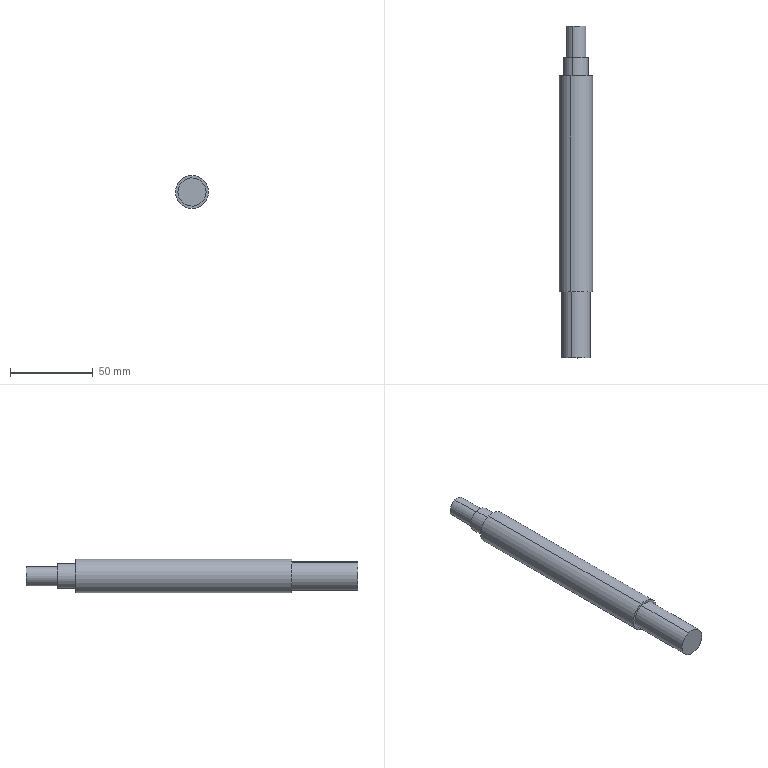Component | SolidWorks | CenterAxis-1 | 1 solid | 13 faces | box 20 x 200 x 20 mm | volume 54013 mm3 | cylinder 8 | plane 5 | commonest cylinder face diameters 12 x2 15 x2 20 x2 17 x2
build123d program:
from build123d import *

# Parameters (mm, degrees)
SKETCH2_R      = 7.5
EXTRUDE1_DEPTH = 11


with BuildPart() as part:
    # Sketch1 → Revolve1 (revolve)
    with BuildSketch(Plane.XY, mode=Mode.PRIVATE) as revolve1_sk:
        Polygon((0, 86.08), (8.5, 86.08), (8.5, 46.08), (10, 46.08), (10, -83.92), (6, -83.92), (6, -113.92), (0, -113.92), align=None)
    revolve(revolve1_sk.sketch.rotate(Axis((0, 0, 0), (0, 1, 0)), 90), axis=Axis((0, 0, 0), (0, 1, 0)))

    # Sketch2 → Extrude1 (add)
    with BuildSketch(Plane.XZ.offset(83.92)):
        with Locations(Location((0, 0, 0), (0, 0, 270))):
            Circle(SKETCH2_R)
    extrude(amount=EXTRUDE1_DEPTH)


solid = part.part

# Placed as in the assembly
solid = solid.moved(Location((-164.784, 362.063, 4), (180, 0, 0)))
STEP:
#1=COLOUR_RGB('',0.7922,0.8196,0.9333);
#2=FILL_AREA_STYLE_COLOUR('',#1);
#3=FILL_AREA_STYLE('',(#2));
#4=SURFACE_STYLE_FILL_AREA(#3);
#5=SURFACE_SIDE_STYLE('',(#4));
#6=SURFACE_STYLE_USAGE(.BOTH.,#5);
#7=PRESENTATION_STYLE_ASSIGNMENT((#6));
#8=CARTESIAN_POINT('',(-6.563,17.991,0.3814));
#9=VERTEX_POINT('',#8);
#10=CARTESIAN_POINT('',(-6.412,17.991,-0.06641));
#11=VERTEX_POINT('',#10);
#12=CARTESIAN_POINT('',(-6.488,17.991,0.1575));
#13=DIRECTION('',(0.,-1.,0.));
#14=DIRECTION('',(0.3188,0.,-0.9478));
#15=AXIS2_PLACEMENT_3D('',#12,#13,#14);
#16=CIRCLE('',#15,0.2362);
#17=EDGE_CURVE('',#9,#11,#16,.T.);
#18=ORIENTED_EDGE('',*,*,#17,.F.);
#19=CARTESIAN_POINT('',(-6.563,18.74,0.3814));
#20=VERTEX_POINT('',#19);
#21=CARTESIAN_POINT('',(-6.563,14.254,0.3814));
#22=DIRECTION('',(-0.,1.,-0.));
#23=VECTOR('',#22,39.37);
#24=LINE('',#21,#23);
#25=EDGE_CURVE('',#9,#20,#24,.T.);
#26=ORIENTED_EDGE('',*,*,#25,.T.);
#27=CARTESIAN_POINT('',(-6.412,18.74,-0.06641));
#28=VERTEX_POINT('',#27);
#29=CARTESIAN_POINT('',(-6.488,18.74,0.1575));
#30=DIRECTION('',(-0.,1.,-0.));
#31=DIRECTION('',(0.3188,0.,-0.9478));
#32=AXIS2_PLACEMENT_3D('',#29,#30,#31);
#33=CIRCLE('',#32,0.2362);
#34=EDGE_CURVE('',#28,#20,#33,.T.);
#35=ORIENTED_EDGE('',*,*,#34,.F.);
#36=CARTESIAN_POINT('',(-6.412,14.254,-0.06641));
#37=DIRECTION('',(-0.,1.,-0.));
#38=VECTOR('',#37,39.37);
#39=LINE('',#36,#38);
#40=EDGE_CURVE('',#11,#28,#39,.T.);
#41=ORIENTED_EDGE('',*,*,#40,.F.);
#42=EDGE_LOOP('',(#18,#26,#35,#41));
#43=FACE_OUTER_BOUND('',#42,.T.);
#44=CARTESIAN_POINT('',(-6.488,14.254,0.1575));
#45=DIRECTION('',(-0.,1.,-0.));
#46=DIRECTION('',(0.3188,0.,-0.9478));
#47=AXIS2_PLACEMENT_3D('',#44,#45,#46);
#48=CYLINDRICAL_SURFACE('',#47,0.2362);
#49=ADVANCED_FACE('',(#43),#48,.T.);
#50=CARTESIAN_POINT('',(-6.393,17.991,-0.1224));
#51=VERTEX_POINT('',#50);
#52=CARTESIAN_POINT('',(-6.582,17.991,0.4373));
#53=VERTEX_POINT('',#52);
#54=CARTESIAN_POINT('',(-6.488,17.991,0.1575));
#55=DIRECTION('',(-0.,1.,-0.));
#56=DIRECTION('',(0.3188,0.,-0.9478));
#57=AXIS2_PLACEMENT_3D('',#54,#55,#56);
#58=CIRCLE('',#57,0.2953);
#59=EDGE_CURVE('',#51,#53,#58,.T.);
#60=ORIENTED_EDGE('',*,*,#59,.F.);
#61=CARTESIAN_POINT('',(-6.393,17.558,-0.1224));
#62=VERTEX_POINT('',#61);
#63=CARTESIAN_POINT('',(-6.393,17.991,-0.1224));
#64=DIRECTION('',(0.,-1.,0.));
#65=VECTOR('',#64,39.37);
#66=LINE('',#63,#65);
#67=EDGE_CURVE('',#51,#62,#66,.T.);
#68=ORIENTED_EDGE('',*,*,#67,.T.);
#69=CARTESIAN_POINT('',(-6.582,17.558,0.4373));
#70=VERTEX_POINT('',#69);
#71=CARTESIAN_POINT('',(-6.488,17.558,0.1575));
#72=DIRECTION('',(-0.,1.,-0.));
#73=DIRECTION('',(0.3188,0.,-0.9478));
#74=AXIS2_PLACEMENT_3D('',#71,#72,#73);
#75=CIRCLE('',#74,0.2953);
#76=EDGE_CURVE('',#62,#70,#75,.T.);
#77=ORIENTED_EDGE('',*,*,#76,.T.);
#78=CARTESIAN_POINT('',(-6.582,17.991,0.4373));
#79=DIRECTION('',(0.,-1.,0.));
#80=VECTOR('',#79,39.37);
#81=LINE('',#78,#80);
#82=EDGE_CURVE('',#53,#70,#81,.T.);
#83=ORIENTED_EDGE('',*,*,#82,.F.);
#84=EDGE_LOOP('',(#60,#68,#77,#83));
#85=FACE_OUTER_BOUND('',#84,.T.);
#86=CARTESIAN_POINT('',(-6.488,17.991,0.1575));
#87=DIRECTION('',(0.,-1.,0.));
#88=DIRECTION('',(-0.3188,0.,0.9478));
#89=AXIS2_PLACEMENT_3D('',#86,#87,#88);
#90=CYLINDRICAL_SURFACE('',#89,0.2953);
#91=ADVANCED_FACE('',(#85),#90,.T.);
#92=CARTESIAN_POINT('',(-6.362,12.44,-0.2157));
#93=VERTEX_POINT('',#92);
#94=CARTESIAN_POINT('',(-6.613,12.44,0.5306));
#95=VERTEX_POINT('',#94);
#96=CARTESIAN_POINT('',(-6.488,12.44,0.1575));
#97=DIRECTION('',(-0.,1.,-0.));
#98=DIRECTION('',(0.3188,0.,-0.9478));
#99=AXIS2_PLACEMENT_3D('',#96,#97,#98);
#100=CIRCLE('',#99,0.3937);
#101=EDGE_CURVE('',#93,#95,#100,.T.);
#102=ORIENTED_EDGE('',*,*,#101,.T.);
#103=CARTESIAN_POINT('',(-6.613,17.558,0.5306));
#104=VERTEX_POINT('',#103);
#105=CARTESIAN_POINT('',(-6.613,14.254,0.5306));
#106=DIRECTION('',(-0.,1.,-0.));
#107=VECTOR('',#106,39.37);
#108=LINE('',#105,#107);
#109=EDGE_CURVE('',#95,#104,#108,.T.);
#110=ORIENTED_EDGE('',*,*,#109,.T.);
#111=CARTESIAN_POINT('',(-6.362,17.558,-0.2157));
#112=VERTEX_POINT('',#111);
#113=CARTESIAN_POINT('',(-6.488,17.558,0.1575));
#114=DIRECTION('',(-0.,1.,-0.));
#115=DIRECTION('',(0.3188,0.,-0.9478));
#116=AXIS2_PLACEMENT_3D('',#113,#114,#115);
#117=CIRCLE('',#116,0.3937);
#118=EDGE_CURVE('',#112,#104,#117,.T.);
#119=ORIENTED_EDGE('',*,*,#118,.F.);
#120=CARTESIAN_POINT('',(-6.362,14.254,-0.2157));
#121=DIRECTION('',(-0.,1.,-0.));
#122=VECTOR('',#121,39.37);
#123=LINE('',#120,#122);
#124=EDGE_CURVE('',#93,#112,#123,.T.);
#125=ORIENTED_EDGE('',*,*,#124,.F.);
#126=EDGE_LOOP('',(#102,#110,#119,#125));
#127=FACE_OUTER_BOUND('',#126,.T.);
#128=CARTESIAN_POINT('',(-6.488,14.254,0.1575));
#129=DIRECTION('',(-0.,1.,-0.));
#130=DIRECTION('',(0.3188,0.,-0.9478));
#131=AXIS2_PLACEMENT_3D('',#128,#129,#130);
#132=CYLINDRICAL_SURFACE('',#131,0.3937);
#133=ADVANCED_FACE('',(#127),#132,.T.);
#134=CARTESIAN_POINT('',(-6.381,10.865,-0.1597));
#135=VERTEX_POINT('',#134);
#136=CARTESIAN_POINT('',(-6.594,10.865,0.4747));
#137=VERTEX_POINT('',#136);
#138=CARTESIAN_POINT('',(-6.488,10.865,0.1575));
#139=DIRECTION('',(-0.,1.,-0.));
#140=DIRECTION('',(0.3188,0.,-0.9478));
#141=AXIS2_PLACEMENT_3D('',#138,#139,#140);
#142=CIRCLE('',#141,0.3346);
#143=EDGE_CURVE('',#135,#137,#142,.T.);
#144=ORIENTED_EDGE('',*,*,#143,.T.);
#145=CARTESIAN_POINT('',(-6.594,12.44,0.4747));
#146=VERTEX_POINT('',#145);
#147=CARTESIAN_POINT('',(-6.594,14.254,0.4747));
#148=DIRECTION('',(-0.,1.,-0.));
#149=VECTOR('',#148,39.37);
#150=LINE('',#147,#149);
#151=EDGE_CURVE('',#137,#146,#150,.T.);
#152=ORIENTED_EDGE('',*,*,#151,.T.);
#153=CARTESIAN_POINT('',(-6.381,12.44,-0.1597));
#154=VERTEX_POINT('',#153);
#155=CARTESIAN_POINT('',(-6.488,12.44,0.1575));
#156=DIRECTION('',(-0.,1.,-0.));
#157=DIRECTION('',(0.3188,0.,-0.9478));
#158=AXIS2_PLACEMENT_3D('',#155,#156,#157);
#159=CIRCLE('',#158,0.3346);
#160=EDGE_CURVE('',#154,#146,#159,.T.);
#161=ORIENTED_EDGE('',*,*,#160,.F.);
#162=CARTESIAN_POINT('',(-6.381,14.254,-0.1597));
#163=DIRECTION('',(-0.,1.,-0.));
#164=VECTOR('',#163,39.37);
#165=LINE('',#162,#164);
#166=EDGE_CURVE('',#135,#154,#165,.T.);
#167=ORIENTED_EDGE('',*,*,#166,.F.);
#168=EDGE_LOOP('',(#144,#152,#161,#167));
#169=FACE_OUTER_BOUND('',#168,.T.);
#170=CARTESIAN_POINT('',(-6.488,14.254,0.1575));
#171=DIRECTION('',(-0.,1.,-0.));
#172=DIRECTION('',(0.3188,0.,-0.9478));
#173=AXIS2_PLACEMENT_3D('',#170,#171,#172);
#174=CYLINDRICAL_SURFACE('',#173,0.3346);
#175=ADVANCED_FACE('',(#169),#174,.T.);
#176=ORIENTED_EDGE('',*,*,#118,.T.);
#177=CARTESIAN_POINT('',(-6.488,17.558,0.1575));
#178=DIRECTION('',(-0.,1.,-0.));
#179=DIRECTION('',(0.3188,0.,-0.9478));
#180=AXIS2_PLACEMENT_3D('',#177,#178,#179);
#181=CIRCLE('',#180,0.3937);
#182=EDGE_CURVE('',#104,#112,#181,.T.);
#183=ORIENTED_EDGE('',*,*,#182,.T.);
#184=EDGE_LOOP('',(#176,#183));
#185=FACE_OUTER_BOUND('',#184,.T.);
#186=CARTESIAN_POINT('',(-6.488,17.558,0.1575));
#187=DIRECTION('',(-0.,1.,-0.));
#188=DIRECTION('',(0.3188,0.,-0.9478));
#189=AXIS2_PLACEMENT_3D('',#186,#187,#188);
#190=CIRCLE('',#189,0.2953);
#191=EDGE_CURVE('',#70,#62,#190,.T.);
#192=ORIENTED_EDGE('',*,*,#191,.F.);
#193=ORIENTED_EDGE('',*,*,#76,.F.);
#194=EDGE_LOOP('',(#192,#193));
#195=FACE_BOUND('',#194,.T.);
#196=CARTESIAN_POINT('',(-6.861,17.558,0.03195));
#197=DIRECTION('',(-0.,1.,-0.));
#198=DIRECTION('',(0.3188,0.,-0.9478));
#199=AXIS2_PLACEMENT_3D('',#196,#197,#198);
#200=PLANE('',#199);
#201=ADVANCED_FACE('',(#185,#195),#200,.T.);
#202=ORIENTED_EDGE('',*,*,#143,.F.);
#203=CARTESIAN_POINT('',(-6.488,10.865,0.1575));
#204=DIRECTION('',(-0.,1.,-0.));
#205=DIRECTION('',(0.3188,0.,-0.9478));
#206=AXIS2_PLACEMENT_3D('',#203,#204,#205);
#207=CIRCLE('',#206,0.3346);
#208=EDGE_CURVE('',#137,#135,#207,.T.);
#209=ORIENTED_EDGE('',*,*,#208,.F.);
#210=EDGE_LOOP('',(#202,#209));
#211=FACE_OUTER_BOUND('',#210,.T.);
#212=CARTESIAN_POINT('',(-6.488,10.865,0.1575));
#213=DIRECTION('',(0.,-1.,0.));
#214=DIRECTION('',(-0.3188,-0.,0.9478));
#215=AXIS2_PLACEMENT_3D('',#212,#213,#214);
#216=PLANE('',#215);
#217=ADVANCED_FACE('',(#211),#216,.T.);
#218=ORIENTED_EDGE('',*,*,#151,.F.);
#219=ORIENTED_EDGE('',*,*,#208,.T.);
#220=ORIENTED_EDGE('',*,*,#166,.T.);
#221=CARTESIAN_POINT('',(-6.488,12.44,0.1575));
#222=DIRECTION('',(-0.,1.,-0.));
#223=DIRECTION('',(0.3188,0.,-0.9478));
#224=AXIS2_PLACEMENT_3D('',#221,#222,#223);
#225=CIRCLE('',#224,0.3346);
#226=EDGE_CURVE('',#146,#154,#225,.T.);
#227=ORIENTED_EDGE('',*,*,#226,.F.);
#228=EDGE_LOOP('',(#218,#219,#220,#227));
#229=FACE_OUTER_BOUND('',#228,.T.);
#230=CARTESIAN_POINT('',(-6.488,14.254,0.1575));
#231=DIRECTION('',(-0.,1.,-0.));
#232=DIRECTION('',(0.3188,0.,-0.9478));
#233=AXIS2_PLACEMENT_3D('',#230,#231,#232);
#234=CYLINDRICAL_SURFACE('',#233,0.3346);
#235=ADVANCED_FACE('',(#229),#234,.T.);
#236=ORIENTED_EDGE('',*,*,#160,.T.);
#237=ORIENTED_EDGE('',*,*,#226,.T.);
#238=EDGE_LOOP('',(#236,#237));
#239=FACE_BOUND('',#238,.T.);
#240=ORIENTED_EDGE('',*,*,#101,.F.);
#241=CARTESIAN_POINT('',(-6.488,12.44,0.1575));
#242=DIRECTION('',(-0.,1.,-0.));
#243=DIRECTION('',(0.3188,0.,-0.9478));
#244=AXIS2_PLACEMENT_3D('',#241,#242,#243);
#245=CIRCLE('',#244,0.3937);
#246=EDGE_CURVE('',#95,#93,#245,.T.);
#247=ORIENTED_EDGE('',*,*,#246,.F.);
#248=EDGE_LOOP('',(#240,#247));
#249=FACE_OUTER_BOUND('',#248,.T.);
#250=CARTESIAN_POINT('',(-6.805,12.44,0.05078));
#251=DIRECTION('',(0.,-1.,0.));
#252=DIRECTION('',(-0.3188,-0.,0.9478));
#253=AXIS2_PLACEMENT_3D('',#250,#251,#252);
#254=PLANE('',#253);
#255=ADVANCED_FACE('',(#239,#249),#254,.T.);
#256=ORIENTED_EDGE('',*,*,#109,.F.);
#257=ORIENTED_EDGE('',*,*,#246,.T.);
#258=ORIENTED_EDGE('',*,*,#124,.T.);
#259=ORIENTED_EDGE('',*,*,#182,.F.);
#260=EDGE_LOOP('',(#256,#257,#258,#259));
#261=FACE_OUTER_BOUND('',#260,.T.);
#262=CARTESIAN_POINT('',(-6.488,14.254,0.1575));
#263=DIRECTION('',(-0.,1.,-0.));
#264=DIRECTION('',(0.3188,0.,-0.9478));
#265=AXIS2_PLACEMENT_3D('',#262,#263,#264);
#266=CYLINDRICAL_SURFACE('',#265,0.3937);
#267=ADVANCED_FACE('',(#261),#266,.T.);
#268=ORIENTED_EDGE('',*,*,#67,.F.);
#269=CARTESIAN_POINT('',(-6.488,17.991,0.1575));
#270=DIRECTION('',(-0.,1.,-0.));
#271=DIRECTION('',(0.3188,0.,-0.9478));
#272=AXIS2_PLACEMENT_3D('',#269,#270,#271);
#273=CIRCLE('',#272,0.2953);
#274=EDGE_CURVE('',#53,#51,#273,.T.);
#275=ORIENTED_EDGE('',*,*,#274,.F.);
#276=ORIENTED_EDGE('',*,*,#82,.T.);
#277=ORIENTED_EDGE('',*,*,#191,.T.);
#278=EDGE_LOOP('',(#268,#275,#276,#277));
#279=FACE_OUTER_BOUND('',#278,.T.);
#280=CARTESIAN_POINT('',(-6.488,17.991,0.1575));
#281=DIRECTION('',(0.,-1.,0.));
#282=DIRECTION('',(-0.3188,0.,0.9478));
#283=AXIS2_PLACEMENT_3D('',#280,#281,#282);
#284=CYLINDRICAL_SURFACE('',#283,0.2953);
#285=ADVANCED_FACE('',(#279),#284,.T.);
#286=CARTESIAN_POINT('',(-6.488,17.991,0.1575));
#287=DIRECTION('',(0.,-1.,0.));
#288=DIRECTION('',(0.3188,0.,-0.9478));
#289=AXIS2_PLACEMENT_3D('',#286,#287,#288);
#290=CIRCLE('',#289,0.2362);
#291=EDGE_CURVE('',#11,#9,#290,.T.);
#292=ORIENTED_EDGE('',*,*,#291,.T.);
#293=ORIENTED_EDGE('',*,*,#17,.T.);
#294=EDGE_LOOP('',(#292,#293));
#295=FACE_BOUND('',#294,.T.);
#296=ORIENTED_EDGE('',*,*,#274,.T.);
#297=ORIENTED_EDGE('',*,*,#59,.T.);
#298=EDGE_LOOP('',(#296,#297));
#299=FACE_OUTER_BOUND('',#298,.T.);
#300=CARTESIAN_POINT('',(-6.488,17.991,0.1575));
#301=DIRECTION('',(-0.,1.,-0.));
#302=DIRECTION('',(0.3188,0.,-0.9478));
#303=AXIS2_PLACEMENT_3D('',#300,#301,#302);
#304=PLANE('',#303);
#305=ADVANCED_FACE('',(#295,#299),#304,.T.);
#306=ORIENTED_EDGE('',*,*,#34,.T.);
#307=CARTESIAN_POINT('',(-6.488,18.74,0.1575));
#308=DIRECTION('',(-0.,1.,-0.));
#309=DIRECTION('',(0.3188,0.,-0.9478));
#310=AXIS2_PLACEMENT_3D('',#307,#308,#309);
#311=CIRCLE('',#310,0.2362);
#312=EDGE_CURVE('',#20,#28,#311,.T.);
#313=ORIENTED_EDGE('',*,*,#312,.T.);
#314=EDGE_LOOP('',(#306,#313));
#315=FACE_OUTER_BOUND('',#314,.T.);
#316=CARTESIAN_POINT('',(-6.711,18.74,0.08216));
#317=DIRECTION('',(-0.,1.,-0.));
#318=DIRECTION('',(0.3188,0.,-0.9478));
#319=AXIS2_PLACEMENT_3D('',#316,#317,#318);
#320=PLANE('',#319);
#321=ADVANCED_FACE('',(#315),#320,.T.);
#322=ORIENTED_EDGE('',*,*,#25,.F.);
#323=ORIENTED_EDGE('',*,*,#291,.F.);
#324=ORIENTED_EDGE('',*,*,#40,.T.);
#325=ORIENTED_EDGE('',*,*,#312,.F.);
#326=EDGE_LOOP('',(#322,#323,#324,#325));
#327=FACE_OUTER_BOUND('',#326,.T.);
#328=CARTESIAN_POINT('',(-6.488,14.254,0.1575));
#329=DIRECTION('',(-0.,1.,-0.));
#330=DIRECTION('',(0.3188,0.,-0.9478));
#331=AXIS2_PLACEMENT_3D('',#328,#329,#330);
#332=CYLINDRICAL_SURFACE('',#331,0.2362);
#333=ADVANCED_FACE('',(#327),#332,.T.);
#334=CLOSED_SHELL('',(#49,#91,#133,#175,#201,#217,#235,#255,#267,#285,#305,#321,#333));
#335=MANIFOLD_SOLID_BREP('',#334);
#336=STYLED_ITEM('',(#7),#335);
#337=PRESENTATION_LAYER_ASSIGNMENT('','',(#336));
#338=CARTESIAN_POINT('',(0.,0.,0.));
#339=DIRECTION('',(0.,0.,1.));
#340=DIRECTION('',(1.,0.,0.));
#341=AXIS2_PLACEMENT_3D('',#338,#339,#340);
#342=(LENGTH_UNIT()NAMED_UNIT(*)SI_UNIT($,.METRE.));
#343=LENGTH_MEASURE_WITH_UNIT(LENGTH_MEASURE(0.0254),#342);
#344=DIMENSIONAL_EXPONENTS(1.,0.,0.,0.,0.,0.,0.);
#345=(CONVERSION_BASED_UNIT('',#343)LENGTH_UNIT()NAMED_UNIT(#344));
#346=UNCERTAINTY_MEASURE_WITH_UNIT(LENGTH_MEASURE(0.00001),#345,'','');
#347=(NAMED_UNIT(*)PLANE_ANGLE_UNIT()SI_UNIT($,.RADIAN.));
#348=(NAMED_UNIT(*)SI_UNIT($,.STERADIAN.)SOLID_ANGLE_UNIT());
#349=(GEOMETRIC_REPRESENTATION_CONTEXT(3)GLOBAL_UNCERTAINTY_ASSIGNED_CONTEXT((#346))GLOBAL_UNIT_ASSIGNED_CONTEXT((#345,#347,#348))REPRESENTATION_CONTEXT('',''));
#350=ADVANCED_BREP_SHAPE_REPRESENTATION('',(#335,#341),#349);
#351=(LENGTH_UNIT()NAMED_UNIT(*)SI_UNIT($,.METRE.));
#352=LENGTH_MEASURE_WITH_UNIT(LENGTH_MEASURE(0.0254),#351);
#353=DIMENSIONAL_EXPONENTS(1.,0.,0.,0.,0.,0.,0.);
#354=(CONVERSION_BASED_UNIT('',#352)LENGTH_UNIT()NAMED_UNIT(#353));
#355=UNCERTAINTY_MEASURE_WITH_UNIT(LENGTH_MEASURE(0.00001),#354,'','');
#356=(NAMED_UNIT(*)PLANE_ANGLE_UNIT()SI_UNIT($,.RADIAN.));
#357=(NAMED_UNIT(*)SI_UNIT($,.STERADIAN.)SOLID_ANGLE_UNIT());
#358=(GEOMETRIC_REPRESENTATION_CONTEXT(3)GLOBAL_UNCERTAINTY_ASSIGNED_CONTEXT((#355))GLOBAL_UNIT_ASSIGNED_CONTEXT((#354,#356,#357))REPRESENTATION_CONTEXT('',''));
#359=MECHANICAL_DESIGN_GEOMETRIC_PRESENTATION_REPRESENTATION('',(#336),#358);